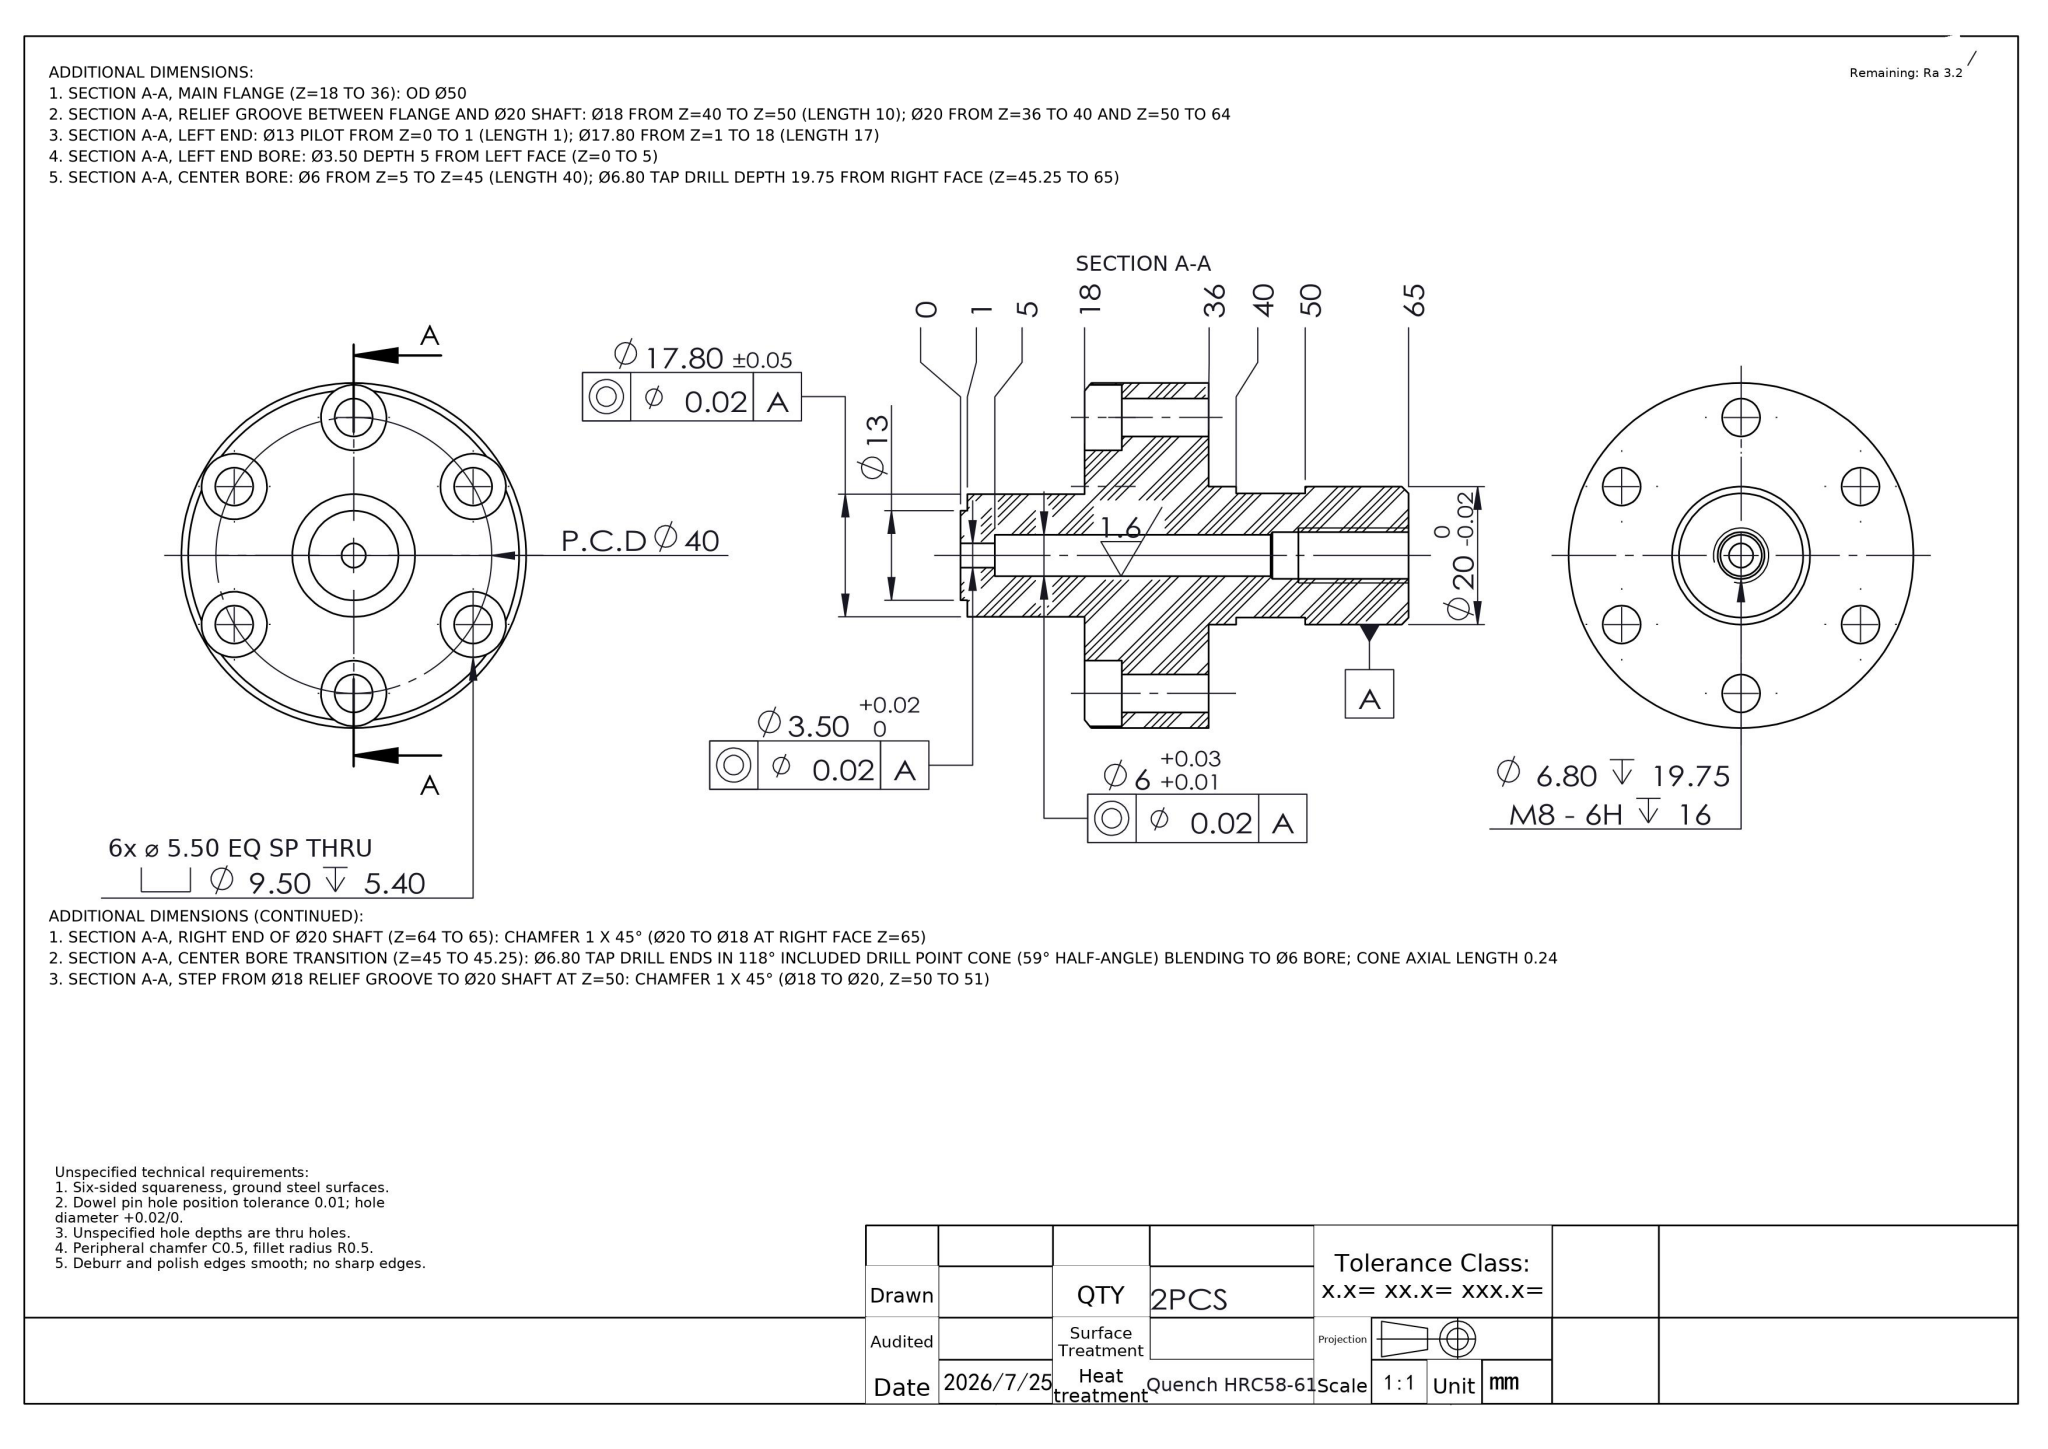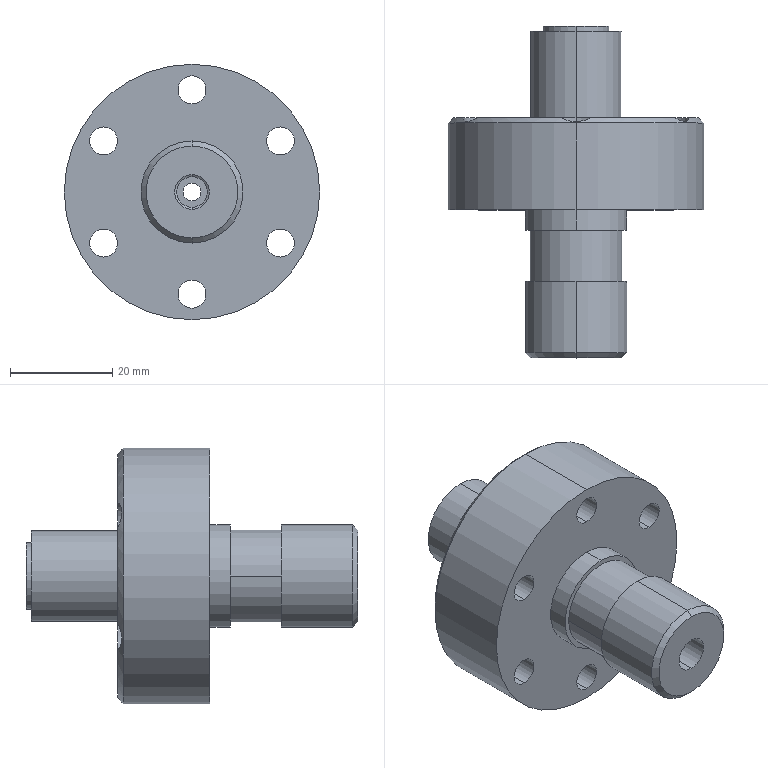Part | NX | mm | 1 solid | 62 faces | box 50 x 65 x 50 mm | volume 42120 mm3 | cylinder 42 | plane 14 | cone 6 | commonest cylinder face diameters 9.5 x12 5.5 x12 20 x4 6.8 x2 3.5 x2 6 x2 18 x2 17.8 x2